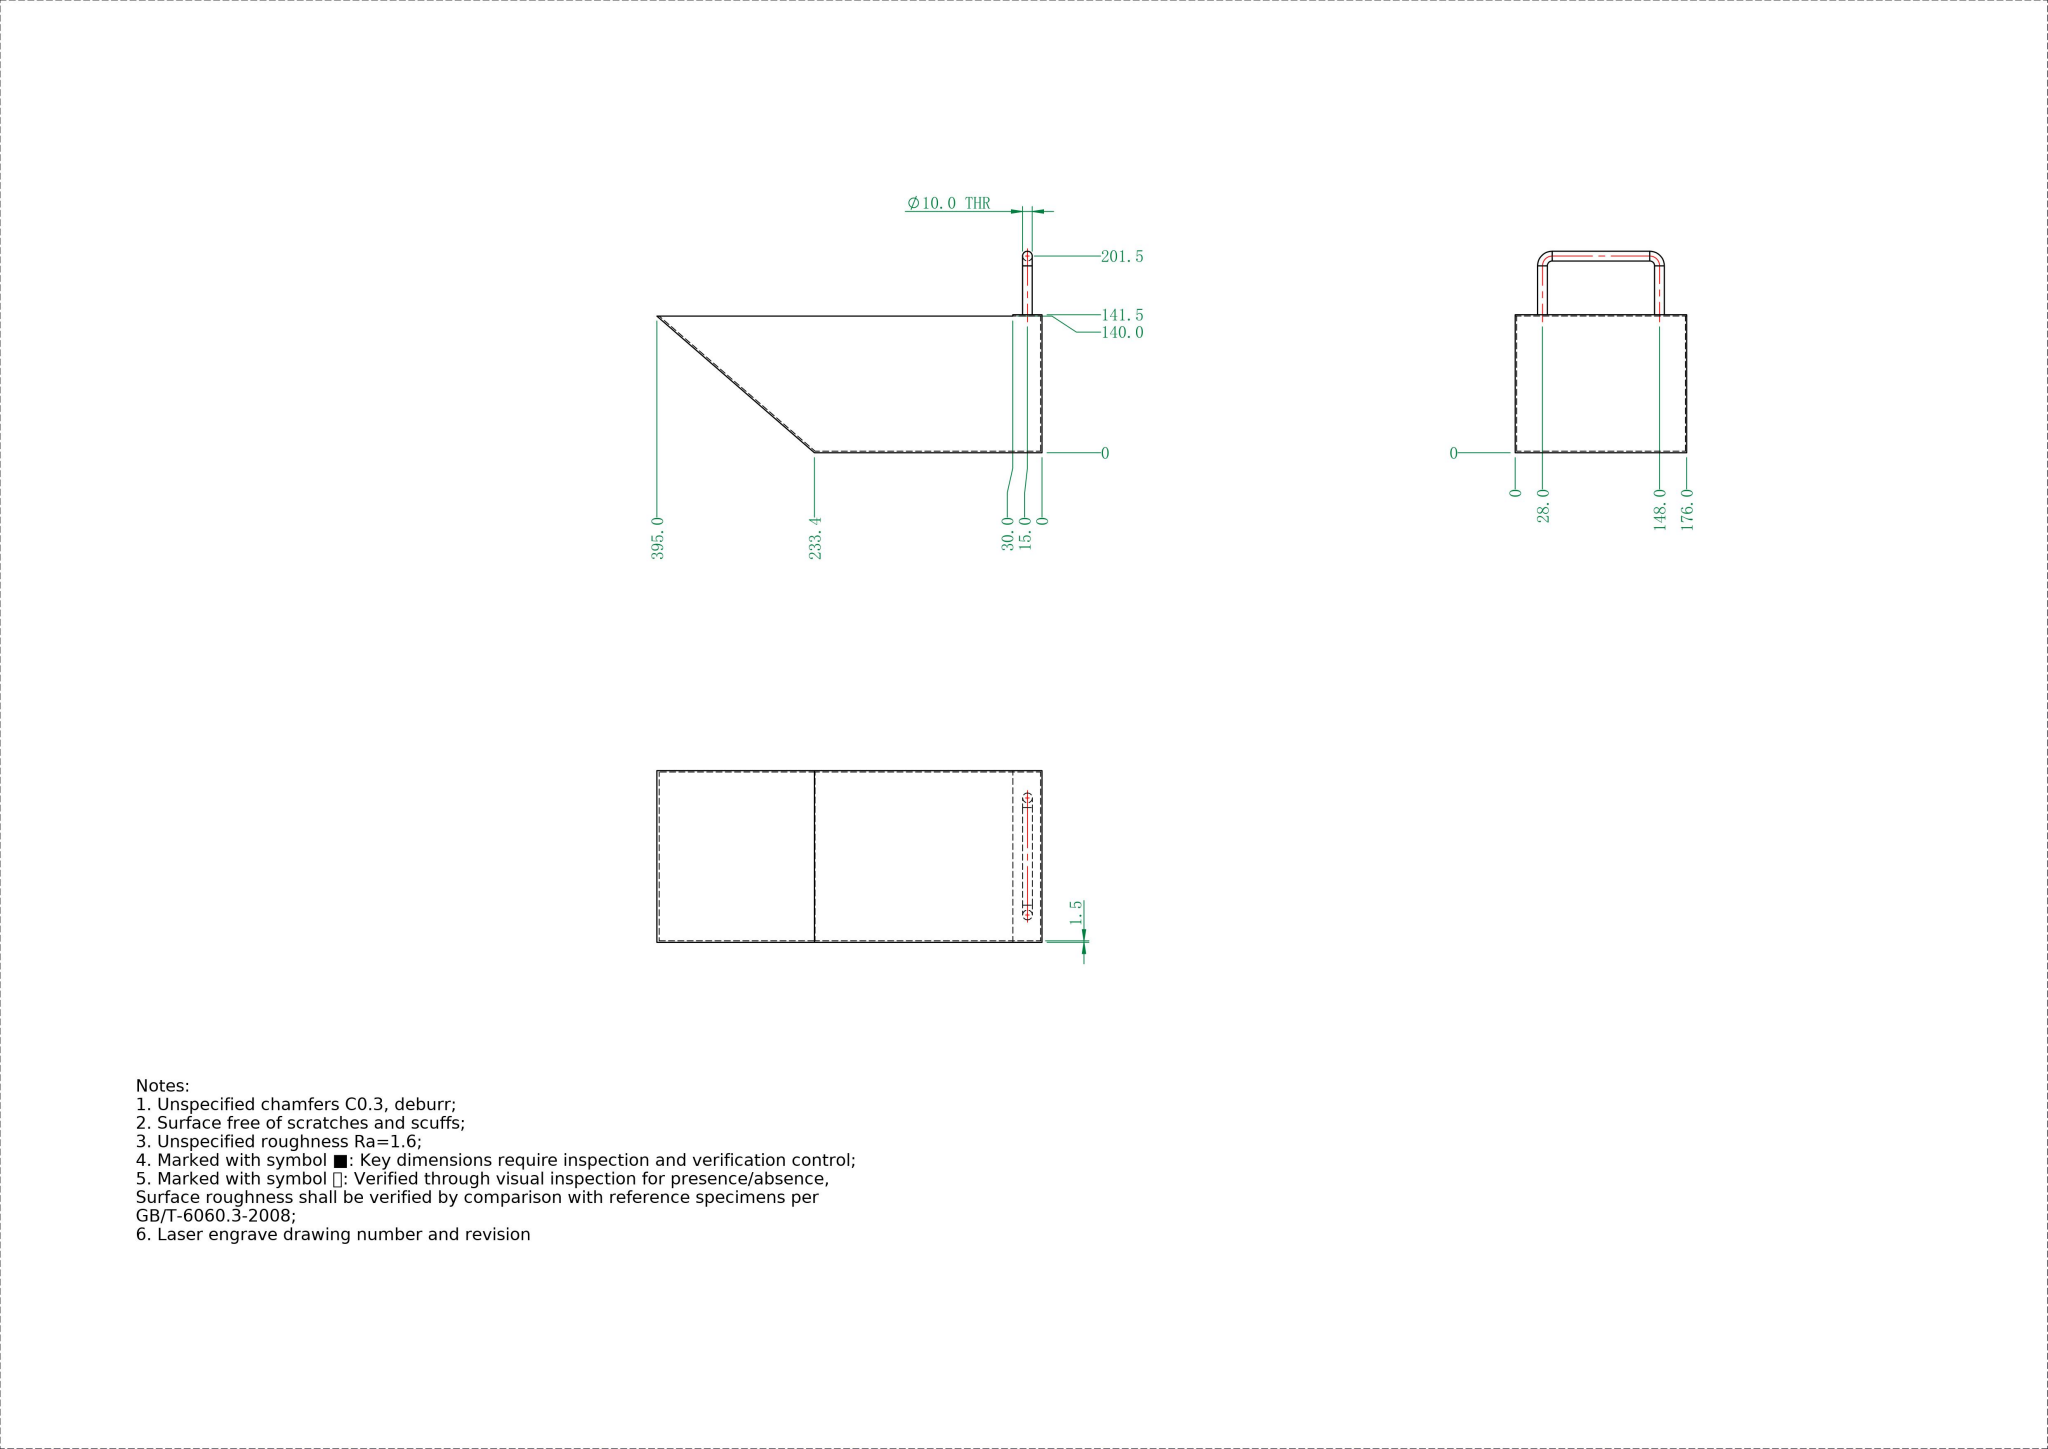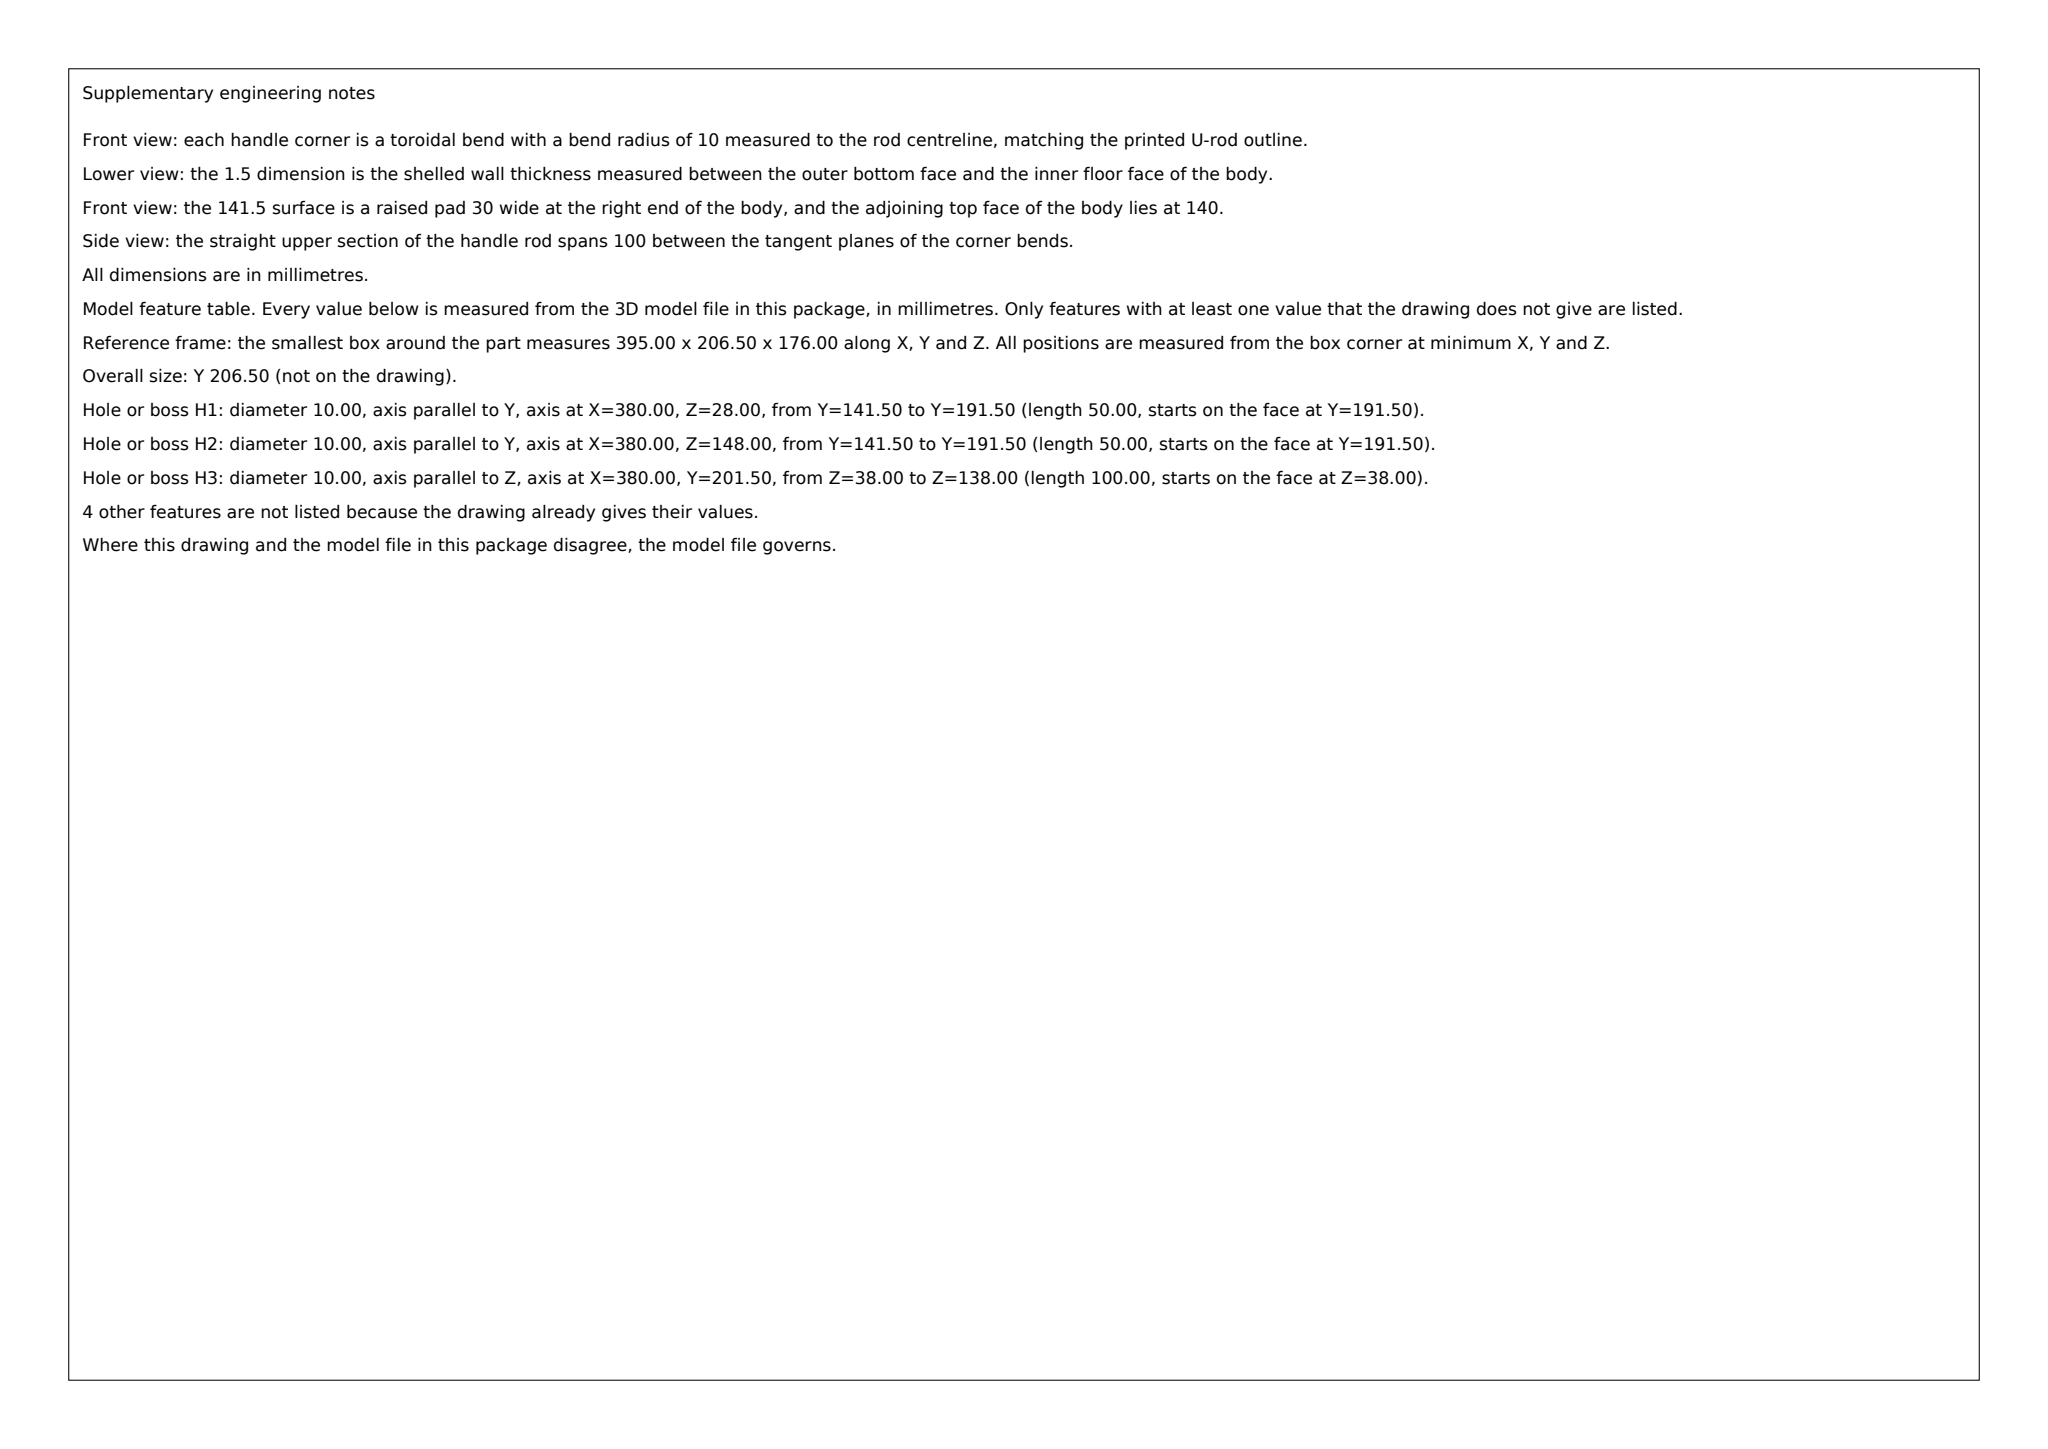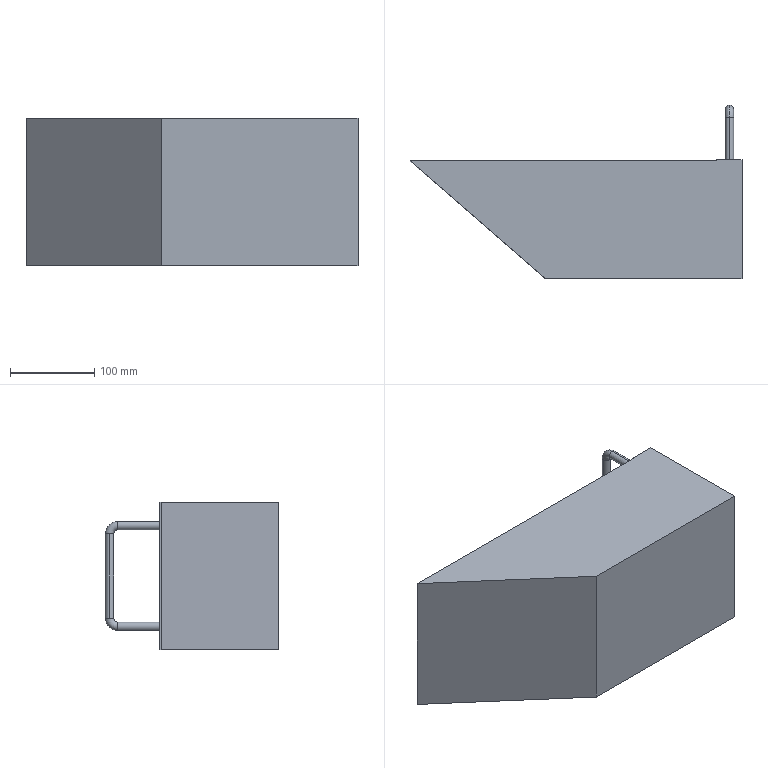Part | SolidWorks | mm | 1 solid | 24 faces | box 395 x 206.5 x 176 mm | volume 309691 mm3 | plane 14 | cylinder 6 | torus 4 | commonest cylinder face diameters 10 x6
Drawing notes:
Ø10.0 THRU | from the solid: Three Ø10.0 cylinders (y-axis at x380,z148 & x380,z28; z-axis at x380,y201.5) all full-depth, dia 10.0
STEP:
#1=CARTESIAN_POINT('',(375.,201.5,38.));
#2=VERTEX_POINT('',#1);
#3=CARTESIAN_POINT('',(380.,206.5,38.));
#4=VERTEX_POINT('',#3);
#5=CARTESIAN_POINT('',(380.,201.5,38.));
#6=DIRECTION('',(0.,0.,-1.));
#7=DIRECTION('',(0.,1.,0.));
#8=AXIS2_PLACEMENT_3D('',#5,#6,#7);
#9=CIRCLE('',#8,5.);
#10=EDGE_CURVE('',#2,#4,#9,.T.);
#11=ORIENTED_EDGE('',*,*,#10,.T.);
#12=CARTESIAN_POINT('',(380.,191.5,23.));
#13=VERTEX_POINT('',#12);
#14=CARTESIAN_POINT('',(380.,191.5,38.));
#15=DIRECTION('',(-1.,0.,0.));
#16=DIRECTION('',(0.,0.,1.));
#17=AXIS2_PLACEMENT_3D('',#14,#15,#16);
#18=CIRCLE('',#17,15.);
#19=EDGE_CURVE('',#4,#13,#18,.T.);
#20=ORIENTED_EDGE('',*,*,#19,.T.);
#21=CARTESIAN_POINT('',(380.,191.5,33.));
#22=VERTEX_POINT('',#21);
#23=CARTESIAN_POINT('',(380.,191.5,28.));
#24=DIRECTION('',(0.,-1.,0.));
#25=DIRECTION('',(0.,0.,-1.));
#26=AXIS2_PLACEMENT_3D('',#23,#24,#25);
#27=CIRCLE('',#26,5.);
#28=EDGE_CURVE('',#22,#13,#27,.T.);
#29=ORIENTED_EDGE('',*,*,#28,.F.);
#30=CARTESIAN_POINT('',(380.,196.5,38.));
#31=VERTEX_POINT('',#30);
#32=CARTESIAN_POINT('',(380.,191.5,38.));
#33=DIRECTION('',(-1.,0.,0.));
#34=DIRECTION('',(0.,0.,1.));
#35=AXIS2_PLACEMENT_3D('',#32,#33,#34);
#36=CIRCLE('',#35,5.);
#37=EDGE_CURVE('',#31,#22,#36,.T.);
#38=ORIENTED_EDGE('',*,*,#37,.F.);
#39=CARTESIAN_POINT('',(380.,201.5,38.));
#40=DIRECTION('',(0.,0.,-1.));
#41=DIRECTION('',(0.,1.,0.));
#42=AXIS2_PLACEMENT_3D('',#39,#40,#41);
#43=CIRCLE('',#42,5.);
#44=EDGE_CURVE('',#31,#2,#43,.T.);
#45=ORIENTED_EDGE('',*,*,#44,.T.);
#46=EDGE_LOOP('',(#11,#20,#29,#38,#45));
#47=FACE_OUTER_BOUND('',#46,.T.);
#48=CARTESIAN_POINT('',(380.,191.5,38.));
#49=DIRECTION('',(-1.,0.,0.));
#50=DIRECTION('',(0.,0.,1.));
#51=AXIS2_PLACEMENT_3D('',#48,#49,#50);
#52=TOROIDAL_SURFACE('',#51,10.,5.);
#53=ADVANCED_FACE('',(#47),#52,.T.);
#54=CARTESIAN_POINT('',(380.,191.5,143.));
#55=VERTEX_POINT('',#54);
#56=CARTESIAN_POINT('',(380.,191.5,153.));
#57=VERTEX_POINT('',#56);
#58=CARTESIAN_POINT('',(380.,191.5,148.));
#59=DIRECTION('',(0.,1.,0.));
#60=DIRECTION('',(0.,0.,1.));
#61=AXIS2_PLACEMENT_3D('',#58,#59,#60);
#62=CIRCLE('',#61,5.);
#63=EDGE_CURVE('',#55,#57,#62,.T.);
#64=ORIENTED_EDGE('',*,*,#63,.T.);
#65=CARTESIAN_POINT('',(380.,206.5,138.));
#66=VERTEX_POINT('',#65);
#67=CARTESIAN_POINT('',(380.,191.5,138.));
#68=DIRECTION('',(-1.,0.,0.));
#69=DIRECTION('',(0.,0.,1.));
#70=AXIS2_PLACEMENT_3D('',#67,#68,#69);
#71=CIRCLE('',#70,15.);
#72=EDGE_CURVE('',#57,#66,#71,.T.);
#73=ORIENTED_EDGE('',*,*,#72,.T.);
#74=CARTESIAN_POINT('',(375.,201.5,138.));
#75=VERTEX_POINT('',#74);
#76=CARTESIAN_POINT('',(380.,201.5,138.));
#77=DIRECTION('',(0.,0.,-1.));
#78=DIRECTION('',(0.,1.,0.));
#79=AXIS2_PLACEMENT_3D('',#76,#77,#78);
#80=CIRCLE('',#79,5.);
#81=EDGE_CURVE('',#75,#66,#80,.T.);
#82=ORIENTED_EDGE('',*,*,#81,.F.);
#83=CARTESIAN_POINT('',(380.,196.5,138.));
#84=VERTEX_POINT('',#83);
#85=CARTESIAN_POINT('',(380.,201.5,138.));
#86=DIRECTION('',(0.,0.,-1.));
#87=DIRECTION('',(0.,1.,0.));
#88=AXIS2_PLACEMENT_3D('',#85,#86,#87);
#89=CIRCLE('',#88,5.);
#90=EDGE_CURVE('',#84,#75,#89,.T.);
#91=ORIENTED_EDGE('',*,*,#90,.F.);
#92=CARTESIAN_POINT('',(380.,191.5,138.));
#93=DIRECTION('',(-1.,0.,0.));
#94=DIRECTION('',(0.,0.,1.));
#95=AXIS2_PLACEMENT_3D('',#92,#93,#94);
#96=CIRCLE('',#95,5.);
#97=EDGE_CURVE('',#55,#84,#96,.T.);
#98=ORIENTED_EDGE('',*,*,#97,.F.);
#99=EDGE_LOOP('',(#64,#73,#82,#91,#98));
#100=FACE_OUTER_BOUND('',#99,.T.);
#101=CARTESIAN_POINT('',(380.,191.5,138.));
#102=DIRECTION('',(-1.,0.,0.));
#103=DIRECTION('',(0.,0.,1.));
#104=AXIS2_PLACEMENT_3D('',#101,#102,#103);
#105=TOROIDAL_SURFACE('',#104,10.,5.);
#106=ADVANCED_FACE('',(#100),#105,.T.);
#107=CARTESIAN_POINT('',(380.,191.5,28.));
#108=DIRECTION('',(0.,-1.,0.));
#109=DIRECTION('',(0.,0.,-1.));
#110=AXIS2_PLACEMENT_3D('',#107,#108,#109);
#111=CIRCLE('',#110,5.);
#112=EDGE_CURVE('',#13,#22,#111,.T.);
#113=ORIENTED_EDGE('',*,*,#112,.T.);
#114=CARTESIAN_POINT('',(380.,141.5,33.));
#115=VERTEX_POINT('',#114);
#116=CARTESIAN_POINT('',(380.,191.5,33.));
#117=DIRECTION('',(0.,-1.,-0.));
#118=VECTOR('',#117,1000.);
#119=LINE('',#116,#118);
#120=EDGE_CURVE('',#22,#115,#119,.T.);
#121=ORIENTED_EDGE('',*,*,#120,.T.);
#122=CARTESIAN_POINT('',(380.,141.5,23.));
#123=VERTEX_POINT('',#122);
#124=CARTESIAN_POINT('',(380.,141.5,28.));
#125=DIRECTION('',(0.,-1.,-0.));
#126=DIRECTION('',(0.,0.,-1.));
#127=AXIS2_PLACEMENT_3D('',#124,#125,#126);
#128=CIRCLE('',#127,5.);
#129=EDGE_CURVE('',#123,#115,#128,.T.);
#130=ORIENTED_EDGE('',*,*,#129,.F.);
#131=CARTESIAN_POINT('',(380.,191.5,23.));
#132=DIRECTION('',(0.,-1.,-0.));
#133=VECTOR('',#132,1000.);
#134=LINE('',#131,#133);
#135=EDGE_CURVE('',#13,#123,#134,.T.);
#136=ORIENTED_EDGE('',*,*,#135,.F.);
#137=EDGE_LOOP('',(#113,#121,#130,#136));
#138=FACE_OUTER_BOUND('',#137,.T.);
#139=CARTESIAN_POINT('',(380.,191.5,28.));
#140=DIRECTION('',(0.,-1.,-0.));
#141=DIRECTION('',(0.,0.,-1.));
#142=AXIS2_PLACEMENT_3D('',#139,#140,#141);
#143=CYLINDRICAL_SURFACE('',#142,5.);
#144=ADVANCED_FACE('',(#138),#143,.T.);
#145=ORIENTED_EDGE('',*,*,#81,.T.);
#146=CARTESIAN_POINT('',(385.,201.5,138.));
#147=VERTEX_POINT('',#146);
#148=CARTESIAN_POINT('',(380.,201.5,138.));
#149=DIRECTION('',(0.,0.,-1.));
#150=DIRECTION('',(0.,1.,0.));
#151=AXIS2_PLACEMENT_3D('',#148,#149,#150);
#152=CIRCLE('',#151,5.);
#153=EDGE_CURVE('',#66,#147,#152,.T.);
#154=ORIENTED_EDGE('',*,*,#153,.T.);
#155=CARTESIAN_POINT('',(385.,201.5,38.));
#156=VERTEX_POINT('',#155);
#157=CARTESIAN_POINT('',(385.,201.5,138.));
#158=DIRECTION('',(0.,0.,-1.));
#159=VECTOR('',#158,1000.);
#160=LINE('',#157,#159);
#161=EDGE_CURVE('',#147,#156,#160,.T.);
#162=ORIENTED_EDGE('',*,*,#161,.T.);
#163=CARTESIAN_POINT('',(380.,201.5,38.));
#164=DIRECTION('',(0.,0.,-1.));
#165=DIRECTION('',(0.,1.,0.));
#166=AXIS2_PLACEMENT_3D('',#163,#164,#165);
#167=CIRCLE('',#166,5.);
#168=EDGE_CURVE('',#4,#156,#167,.T.);
#169=ORIENTED_EDGE('',*,*,#168,.F.);
#170=ORIENTED_EDGE('',*,*,#10,.F.);
#171=CARTESIAN_POINT('',(375.,201.5,138.));
#172=DIRECTION('',(0.,0.,-1.));
#173=VECTOR('',#172,1000.);
#174=LINE('',#171,#173);
#175=EDGE_CURVE('',#75,#2,#174,.T.);
#176=ORIENTED_EDGE('',*,*,#175,.F.);
#177=EDGE_LOOP('',(#145,#154,#162,#169,#170,#176));
#178=FACE_OUTER_BOUND('',#177,.T.);
#179=CARTESIAN_POINT('',(380.,201.5,138.));
#180=DIRECTION('',(0.,0.,-1.));
#181=DIRECTION('',(-1.,0.,0.));
#182=AXIS2_PLACEMENT_3D('',#179,#180,#181);
#183=CYLINDRICAL_SURFACE('',#182,5.);
#184=ADVANCED_FACE('',(#178),#183,.T.);
#185=CARTESIAN_POINT('',(380.,141.5,153.));
#186=VERTEX_POINT('',#185);
#187=CARTESIAN_POINT('',(380.,141.5,143.));
#188=VERTEX_POINT('',#187);
#189=CARTESIAN_POINT('',(380.,141.5,148.));
#190=DIRECTION('',(0.,1.,0.));
#191=DIRECTION('',(0.,0.,1.));
#192=AXIS2_PLACEMENT_3D('',#189,#190,#191);
#193=CIRCLE('',#192,5.);
#194=EDGE_CURVE('',#186,#188,#193,.T.);
#195=ORIENTED_EDGE('',*,*,#194,.T.);
#196=CARTESIAN_POINT('',(380.,141.5,143.));
#197=DIRECTION('',(0.,1.,0.));
#198=VECTOR('',#197,1000.);
#199=LINE('',#196,#198);
#200=EDGE_CURVE('',#188,#55,#199,.T.);
#201=ORIENTED_EDGE('',*,*,#200,.T.);
#202=CARTESIAN_POINT('',(380.,191.5,148.));
#203=DIRECTION('',(0.,1.,0.));
#204=DIRECTION('',(0.,0.,1.));
#205=AXIS2_PLACEMENT_3D('',#202,#203,#204);
#206=CIRCLE('',#205,5.);
#207=EDGE_CURVE('',#57,#55,#206,.T.);
#208=ORIENTED_EDGE('',*,*,#207,.F.);
#209=CARTESIAN_POINT('',(380.,141.5,153.));
#210=DIRECTION('',(0.,1.,0.));
#211=VECTOR('',#210,1000.);
#212=LINE('',#209,#211);
#213=EDGE_CURVE('',#186,#57,#212,.T.);
#214=ORIENTED_EDGE('',*,*,#213,.F.);
#215=EDGE_LOOP('',(#195,#201,#208,#214));
#216=FACE_OUTER_BOUND('',#215,.T.);
#217=CARTESIAN_POINT('',(380.,141.5,148.));
#218=DIRECTION('',(0.,1.,0.));
#219=DIRECTION('',(0.,0.,1.));
#220=AXIS2_PLACEMENT_3D('',#217,#218,#219);
#221=CYLINDRICAL_SURFACE('',#220,5.);
#222=ADVANCED_FACE('',(#216),#221,.T.);
#223=CARTESIAN_POINT('',(395.,141.5,176.));
#224=VERTEX_POINT('',#223);
#225=CARTESIAN_POINT('',(395.,141.5,0.));
#226=VERTEX_POINT('',#225);
#227=CARTESIAN_POINT('',(395.,141.5,0.));
#228=DIRECTION('',(0.,0.,-1.));
#229=VECTOR('',#228,1000.);
#230=LINE('',#227,#229);
#231=EDGE_CURVE('',#224,#226,#230,.T.);
#232=ORIENTED_EDGE('',*,*,#231,.T.);
#233=CARTESIAN_POINT('',(365.,141.5,0.));
#234=VERTEX_POINT('',#233);
#235=CARTESIAN_POINT('',(395.,141.5,0.));
#236=DIRECTION('',(-1.,0.,0.));
#237=VECTOR('',#236,1000.);
#238=LINE('',#235,#237);
#239=EDGE_CURVE('',#226,#234,#238,.T.);
#240=ORIENTED_EDGE('',*,*,#239,.T.);
#241=CARTESIAN_POINT('',(365.,141.5,176.));
#242=VERTEX_POINT('',#241);
#243=CARTESIAN_POINT('',(365.,141.5,0.));
#244=DIRECTION('',(0.,0.,1.));
#245=VECTOR('',#244,1000.);
#246=LINE('',#243,#245);
#247=EDGE_CURVE('',#234,#242,#246,.T.);
#248=ORIENTED_EDGE('',*,*,#247,.T.);
#249=CARTESIAN_POINT('',(395.,141.5,176.));
#250=DIRECTION('',(1.,0.,0.));
#251=VECTOR('',#250,1000.);
#252=LINE('',#249,#251);
#253=EDGE_CURVE('',#242,#224,#252,.T.);
#254=ORIENTED_EDGE('',*,*,#253,.T.);
#255=EDGE_LOOP('',(#232,#240,#248,#254));
#256=FACE_OUTER_BOUND('',#255,.T.);
#257=ORIENTED_EDGE('',*,*,#194,.F.);
#258=CARTESIAN_POINT('',(380.,141.5,148.));
#259=DIRECTION('',(0.,1.,0.));
#260=DIRECTION('',(0.,0.,1.));
#261=AXIS2_PLACEMENT_3D('',#258,#259,#260);
#262=CIRCLE('',#261,5.);
#263=EDGE_CURVE('',#188,#186,#262,.T.);
#264=ORIENTED_EDGE('',*,*,#263,.F.);
#265=EDGE_LOOP('',(#257,#264));
#266=FACE_BOUND('',#265,.T.);
#267=ORIENTED_EDGE('',*,*,#129,.T.);
#268=CARTESIAN_POINT('',(380.,141.5,28.));
#269=DIRECTION('',(0.,-1.,-0.));
#270=DIRECTION('',(0.,0.,-1.));
#271=AXIS2_PLACEMENT_3D('',#268,#269,#270);
#272=CIRCLE('',#271,5.);
#273=EDGE_CURVE('',#115,#123,#272,.T.);
#274=ORIENTED_EDGE('',*,*,#273,.T.);
#275=EDGE_LOOP('',(#267,#274));
#276=FACE_BOUND('',#275,.T.);
#277=CARTESIAN_POINT('',(0.,141.5,0.));
#278=DIRECTION('',(0.,-1.,0.));
#279=DIRECTION('',(0.,0.,-1.));
#280=AXIS2_PLACEMENT_3D('',#277,#278,#279);
#281=PLANE('',#280);
#282=ADVANCED_FACE('',(#256,#266,#276),#281,.F.);
#283=CARTESIAN_POINT('',(365.,140.,0.));
#284=VERTEX_POINT('',#283);
#285=CARTESIAN_POINT('',(365.,140.,1.5));
#286=VERTEX_POINT('',#285);
#287=CARTESIAN_POINT('',(365.,140.,0.));
#288=DIRECTION('',(0.,0.,1.));
#289=VECTOR('',#288,1000.);
#290=LINE('',#287,#289);
#291=EDGE_CURVE('',#284,#286,#290,.T.);
#292=ORIENTED_EDGE('',*,*,#291,.F.);
#293=CARTESIAN_POINT('',(0.,140.,0.));
#294=VERTEX_POINT('',#293);
#295=CARTESIAN_POINT('',(0.,140.,0.));
#296=DIRECTION('',(-1.,0.,0.));
#297=VECTOR('',#296,1000.);
#298=LINE('',#295,#297);
#299=EDGE_CURVE('',#284,#294,#298,.T.);
#300=ORIENTED_EDGE('',*,*,#299,.T.);
#301=CARTESIAN_POINT('',(0.,140.,176.));
#302=VERTEX_POINT('',#301);
#303=CARTESIAN_POINT('',(0.,140.,176.));
#304=DIRECTION('',(0.,0.,-1.));
#305=VECTOR('',#304,1000.);
#306=LINE('',#303,#305);
#307=EDGE_CURVE('',#302,#294,#306,.T.);
#308=ORIENTED_EDGE('',*,*,#307,.F.);
#309=CARTESIAN_POINT('',(365.,140.,176.));
#310=VERTEX_POINT('',#309);
#311=CARTESIAN_POINT('',(0.,140.,176.));
#312=DIRECTION('',(-1.,0.,0.));
#313=VECTOR('',#312,1000.);
#314=LINE('',#311,#313);
#315=EDGE_CURVE('',#310,#302,#314,.T.);
#316=ORIENTED_EDGE('',*,*,#315,.F.);
#317=CARTESIAN_POINT('',(365.,140.,174.5));
#318=VERTEX_POINT('',#317);
#319=CARTESIAN_POINT('',(365.,140.,0.));
#320=DIRECTION('',(0.,0.,1.));
#321=VECTOR('',#320,1000.);
#322=LINE('',#319,#321);
#323=EDGE_CURVE('',#318,#310,#322,.T.);
#324=ORIENTED_EDGE('',*,*,#323,.F.);
#325=CARTESIAN_POINT('',(2.291,140.,174.5));
#326=VERTEX_POINT('',#325);
#327=CARTESIAN_POINT('',(0.,140.,174.5));
#328=DIRECTION('',(-1.,0.,0.));
#329=VECTOR('',#328,1000.);
#330=LINE('',#327,#329);
#331=EDGE_CURVE('',#318,#326,#330,.T.);
#332=ORIENTED_EDGE('',*,*,#331,.T.);
#333=CARTESIAN_POINT('',(2.291,140.,1.5));
#334=VERTEX_POINT('',#333);
#335=CARTESIAN_POINT('',(2.291,140.,-15.));
#336=DIRECTION('',(0.,0.,-1.));
#337=VECTOR('',#336,1000.);
#338=LINE('',#335,#337);
#339=EDGE_CURVE('',#326,#334,#338,.T.);
#340=ORIENTED_EDGE('',*,*,#339,.T.);
#341=CARTESIAN_POINT('',(0.,140.,1.5));
#342=DIRECTION('',(-1.,0.,0.));
#343=VECTOR('',#342,1000.);
#344=LINE('',#341,#343);
#345=EDGE_CURVE('',#286,#334,#344,.T.);
#346=ORIENTED_EDGE('',*,*,#345,.F.);
#347=EDGE_LOOP('',(#292,#300,#308,#316,#324,#332,#340,#346));
#348=FACE_OUTER_BOUND('',#347,.T.);
#349=CARTESIAN_POINT('',(0.,140.,176.));
#350=DIRECTION('',(0.,-1.,0.));
#351=DIRECTION('',(0.,0.,-1.));
#352=AXIS2_PLACEMENT_3D('',#349,#350,#351);
#353=PLANE('',#352);
#354=ADVANCED_FACE('',(#348),#353,.F.);
#355=CARTESIAN_POINT('',(161.563,0.,176.));
#356=VERTEX_POINT('',#355);
#357=CARTESIAN_POINT('',(395.,0.,176.));
#358=VERTEX_POINT('',#357);
#359=CARTESIAN_POINT('',(0.,0.,176.));
#360=DIRECTION('',(1.,0.,0.));
#361=VECTOR('',#360,1000.);
#362=LINE('',#359,#361);
#363=EDGE_CURVE('',#356,#358,#362,.T.);
#364=ORIENTED_EDGE('',*,*,#363,.F.);
#365=CARTESIAN_POINT('',(161.563,0.,0.));
#366=VERTEX_POINT('',#365);
#367=CARTESIAN_POINT('',(161.563,0.,-15.));
#368=DIRECTION('',(0.,0.,1.));
#369=VECTOR('',#368,1000.);
#370=LINE('',#367,#369);
#371=EDGE_CURVE('',#366,#356,#370,.T.);
#372=ORIENTED_EDGE('',*,*,#371,.F.);
#373=CARTESIAN_POINT('',(395.,0.,0.));
#374=VERTEX_POINT('',#373);
#375=CARTESIAN_POINT('',(0.,0.,0.));
#376=DIRECTION('',(1.,0.,0.));
#377=VECTOR('',#376,1000.);
#378=LINE('',#375,#377);
#379=EDGE_CURVE('',#366,#374,#378,.T.);
#380=ORIENTED_EDGE('',*,*,#379,.T.);
#381=CARTESIAN_POINT('',(395.,0.,176.));
#382=DIRECTION('',(0.,0.,-1.));
#383=VECTOR('',#382,1000.);
#384=LINE('',#381,#383);
#385=EDGE_CURVE('',#358,#374,#384,.T.);
#386=ORIENTED_EDGE('',*,*,#385,.F.);
#387=EDGE_LOOP('',(#364,#372,#380,#386));
#388=FACE_OUTER_BOUND('',#387,.T.);
#389=CARTESIAN_POINT('',(0.,0.,176.));
#390=DIRECTION('',(0.,1.,0.));
#391=DIRECTION('',(0.,0.,1.));
#392=AXIS2_PLACEMENT_3D('',#389,#390,#391);
#393=PLANE('',#392);
#394=ADVANCED_FACE('',(#388),#393,.F.);
#395=CARTESIAN_POINT('',(395.,0.,0.));
#396=DIRECTION('',(0.,1.,0.));
#397=VECTOR('',#396,1000.);
#398=LINE('',#395,#397);
#399=EDGE_CURVE('',#374,#226,#398,.T.);
#400=ORIENTED_EDGE('',*,*,#399,.T.);
#401=ORIENTED_EDGE('',*,*,#231,.F.);
#402=CARTESIAN_POINT('',(395.,0.,176.));
#403=DIRECTION('',(0.,1.,0.));
#404=VECTOR('',#403,1000.);
#405=LINE('',#402,#404);
#406=EDGE_CURVE('',#358,#224,#405,.T.);
#407=ORIENTED_EDGE('',*,*,#406,.F.);
#408=ORIENTED_EDGE('',*,*,#385,.T.);
#409=EDGE_LOOP('',(#400,#401,#407,#408));
#410=FACE_OUTER_BOUND('',#409,.T.);
#411=CARTESIAN_POINT('',(395.,0.,176.));
#412=DIRECTION('',(-1.,0.,0.));
#413=DIRECTION('',(0.,0.,1.));
#414=AXIS2_PLACEMENT_3D('',#411,#412,#413);
#415=PLANE('',#414);
#416=ADVANCED_FACE('',(#410),#415,.F.);
#417=ORIENTED_EDGE('',*,*,#406,.T.);
#418=ORIENTED_EDGE('',*,*,#253,.F.);
#419=CARTESIAN_POINT('',(365.,141.5,176.));
#420=DIRECTION('',(0.,-1.,0.));
#421=VECTOR('',#420,1000.);
#422=LINE('',#419,#421);
#423=EDGE_CURVE('',#242,#310,#422,.T.);
#424=ORIENTED_EDGE('',*,*,#423,.T.);
#425=ORIENTED_EDGE('',*,*,#315,.T.);
#426=CARTESIAN_POINT('',(161.563,0.,176.));
#427=DIRECTION('',(-0.7557,0.6549,0.));
#428=VECTOR('',#427,1000.);
#429=LINE('',#426,#428);
#430=EDGE_CURVE('',#356,#302,#429,.T.);
#431=ORIENTED_EDGE('',*,*,#430,.F.);
#432=ORIENTED_EDGE('',*,*,#363,.T.);
#433=EDGE_LOOP('',(#417,#418,#424,#425,#431,#432));
#434=FACE_OUTER_BOUND('',#433,.T.);
#435=CARTESIAN_POINT('',(0.,0.,176.));
#436=DIRECTION('',(0.,0.,-1.));
#437=DIRECTION('',(-1.,0.,0.));
#438=AXIS2_PLACEMENT_3D('',#435,#436,#437);
#439=PLANE('',#438);
#440=ADVANCED_FACE('',(#434),#439,.F.);
#441=CARTESIAN_POINT('',(69.288,79.96,0.));
#442=DIRECTION('',(0.7557,-0.6549,0.));
#443=VECTOR('',#442,1000.);
#444=LINE('',#441,#443);
#445=EDGE_CURVE('',#294,#366,#444,.T.);
#446=ORIENTED_EDGE('',*,*,#445,.F.);
#447=ORIENTED_EDGE('',*,*,#299,.F.);
#448=CARTESIAN_POINT('',(365.,141.5,0.));
#449=DIRECTION('',(0.,-1.,0.));
#450=VECTOR('',#449,1000.);
#451=LINE('',#448,#450);
#452=EDGE_CURVE('',#234,#284,#451,.T.);
#453=ORIENTED_EDGE('',*,*,#452,.F.);
#454=ORIENTED_EDGE('',*,*,#239,.F.);
#455=ORIENTED_EDGE('',*,*,#399,.F.);
#456=ORIENTED_EDGE('',*,*,#379,.F.);
#457=EDGE_LOOP('',(#446,#447,#453,#454,#455,#456));
#458=FACE_OUTER_BOUND('',#457,.T.);
#459=CARTESIAN_POINT('',(0.,0.,0.));
#460=DIRECTION('',(0.,0.,-1.));
#461=DIRECTION('',(-1.,0.,0.));
#462=AXIS2_PLACEMENT_3D('',#459,#460,#461);
#463=PLANE('',#462);
#464=ADVANCED_FACE('',(#458),#463,.T.);
#465=ORIENTED_EDGE('',*,*,#445,.T.);
#466=ORIENTED_EDGE('',*,*,#371,.T.);
#467=ORIENTED_EDGE('',*,*,#430,.T.);
#468=ORIENTED_EDGE('',*,*,#307,.T.);
#469=EDGE_LOOP('',(#465,#466,#467,#468));
#470=FACE_OUTER_BOUND('',#469,.T.);
#471=CARTESIAN_POINT('',(161.563,0.,-15.));
#472=DIRECTION('',(0.6549,0.7557,0.));
#473=DIRECTION('',(-0.7557,0.6549,0.));
#474=AXIS2_PLACEMENT_3D('',#471,#472,#473);
#475=PLANE('',#474);
#476=ADVANCED_FACE('',(#470),#475,.F.);
#477=CARTESIAN_POINT('',(162.123,1.5,174.5));
#478=VERTEX_POINT('',#477);
#479=CARTESIAN_POINT('',(393.5,1.5,174.5));
#480=VERTEX_POINT('',#479);
#481=CARTESIAN_POINT('',(0.,1.5,174.5));
#482=DIRECTION('',(1.,0.,0.));
#483=VECTOR('',#482,1000.);
#484=LINE('',#481,#483);
#485=EDGE_CURVE('',#478,#480,#484,.T.);
#486=ORIENTED_EDGE('',*,*,#485,.T.);
#487=CARTESIAN_POINT('',(393.5,1.5,1.5));
#488=VERTEX_POINT('',#487);
#489=CARTESIAN_POINT('',(393.5,1.5,176.));
#490=DIRECTION('',(0.,0.,-1.));
#491=VECTOR('',#490,1000.);
#492=LINE('',#489,#491);
#493=EDGE_CURVE('',#480,#488,#492,.T.);
#494=ORIENTED_EDGE('',*,*,#493,.T.);
#495=CARTESIAN_POINT('',(162.123,1.5,1.5));
#496=VERTEX_POINT('',#495);
#497=CARTESIAN_POINT('',(0.,1.5,1.5));
#498=DIRECTION('',(1.,0.,0.));
#499=VECTOR('',#498,1000.);
#500=LINE('',#497,#499);
#501=EDGE_CURVE('',#496,#488,#500,.T.);
#502=ORIENTED_EDGE('',*,*,#501,.F.);
#503=CARTESIAN_POINT('',(162.123,1.5,-15.));
#504=DIRECTION('',(0.,0.,1.));
#505=VECTOR('',#504,1000.);
#506=LINE('',#503,#505);
#507=EDGE_CURVE('',#496,#478,#506,.T.);
#508=ORIENTED_EDGE('',*,*,#507,.T.);
#509=EDGE_LOOP('',(#486,#494,#502,#508));
#510=FACE_OUTER_BOUND('',#509,.T.);
#511=CARTESIAN_POINT('',(0.,1.5,176.));
#512=DIRECTION('',(0.,1.,0.));
#513=DIRECTION('',(0.,0.,1.));
#514=AXIS2_PLACEMENT_3D('',#511,#512,#513);
#515=PLANE('',#514);
#516=ADVANCED_FACE('',(#510),#515,.T.);
#517=CARTESIAN_POINT('',(393.5,140.,1.5));
#518=VERTEX_POINT('',#517);
#519=CARTESIAN_POINT('',(393.5,0.,1.5));
#520=DIRECTION('',(0.,1.,0.));
#521=VECTOR('',#520,1000.);
#522=LINE('',#519,#521);
#523=EDGE_CURVE('',#488,#518,#522,.T.);
#524=ORIENTED_EDGE('',*,*,#523,.F.);
#525=ORIENTED_EDGE('',*,*,#493,.F.);
#526=CARTESIAN_POINT('',(393.5,140.,174.5));
#527=VERTEX_POINT('',#526);
#528=CARTESIAN_POINT('',(393.5,0.,174.5));
#529=DIRECTION('',(0.,1.,0.));
#530=VECTOR('',#529,1000.);
#531=LINE('',#528,#530);
#532=EDGE_CURVE('',#480,#527,#531,.T.);
#533=ORIENTED_EDGE('',*,*,#532,.T.);
#534=CARTESIAN_POINT('',(393.5,140.,176.));
#535=DIRECTION('',(0.,0.,-1.));
#536=VECTOR('',#535,1000.);
#537=LINE('',#534,#536);
#538=EDGE_CURVE('',#527,#518,#537,.T.);
#539=ORIENTED_EDGE('',*,*,#538,.T.);
#540=EDGE_LOOP('',(#524,#525,#533,#539));
#541=FACE_OUTER_BOUND('',#540,.T.);
#542=CARTESIAN_POINT('',(393.5,0.,176.));
#543=DIRECTION('',(-1.,0.,0.));
#544=DIRECTION('',(0.,0.,1.));
#545=AXIS2_PLACEMENT_3D('',#542,#543,#544);
#546=PLANE('',#545);
#547=ADVANCED_FACE('',(#541),#546,.T.);
#548=CARTESIAN_POINT('',(0.,140.,174.5));
#549=DIRECTION('',(-1.,0.,0.));
#550=VECTOR('',#549,1000.);
#551=LINE('',#548,#550);
#552=EDGE_CURVE('',#527,#318,#551,.T.);
#553=ORIENTED_EDGE('',*,*,#552,.F.);
#554=ORIENTED_EDGE('',*,*,#532,.F.);
#555=ORIENTED_EDGE('',*,*,#485,.F.);
#556=CARTESIAN_POINT('',(162.546,1.134,174.5));
#557=DIRECTION('',(-0.7557,0.6549,0.));
#558=VECTOR('',#557,1000.);
#559=LINE('',#556,#558);
#560=EDGE_CURVE('',#478,#326,#559,.T.);
#561=ORIENTED_EDGE('',*,*,#560,.T.);
#562=ORIENTED_EDGE('',*,*,#331,.F.);
#563=EDGE_LOOP('',(#553,#554,#555,#561,#562));
#564=FACE_OUTER_BOUND('',#563,.T.);
#565=CARTESIAN_POINT('',(0.,0.,174.5));
#566=DIRECTION('',(0.,0.,-1.));
#567=DIRECTION('',(-1.,0.,0.));
#568=AXIS2_PLACEMENT_3D('',#565,#566,#567);
#569=PLANE('',#568);
#570=ADVANCED_FACE('',(#564),#569,.T.);
#571=CARTESIAN_POINT('',(70.27,81.093,1.5));
#572=DIRECTION('',(0.7557,-0.6549,0.));
#573=VECTOR('',#572,1000.);
#574=LINE('',#571,#573);
#575=EDGE_CURVE('',#334,#496,#574,.T.);
#576=ORIENTED_EDGE('',*,*,#575,.T.);
#577=ORIENTED_EDGE('',*,*,#501,.T.);
#578=ORIENTED_EDGE('',*,*,#523,.T.);
#579=CARTESIAN_POINT('',(0.,140.,1.5));
#580=DIRECTION('',(-1.,0.,0.));
#581=VECTOR('',#580,1000.);
#582=LINE('',#579,#581);
#583=EDGE_CURVE('',#518,#286,#582,.T.);
#584=ORIENTED_EDGE('',*,*,#583,.T.);
#585=ORIENTED_EDGE('',*,*,#345,.T.);
#586=EDGE_LOOP('',(#576,#577,#578,#584,#585));
#587=FACE_OUTER_BOUND('',#586,.T.);
#588=CARTESIAN_POINT('',(0.,0.,1.5));
#589=DIRECTION('',(0.,0.,-1.));
#590=DIRECTION('',(-1.,0.,0.));
#591=AXIS2_PLACEMENT_3D('',#588,#589,#590);
#592=PLANE('',#591);
#593=ADVANCED_FACE('',(#587),#592,.F.);
#594=ORIENTED_EDGE('',*,*,#575,.F.);
#595=ORIENTED_EDGE('',*,*,#339,.F.);
#596=ORIENTED_EDGE('',*,*,#560,.F.);
#597=ORIENTED_EDGE('',*,*,#507,.F.);
#598=EDGE_LOOP('',(#594,#595,#596,#597));
#599=FACE_OUTER_BOUND('',#598,.T.);
#600=CARTESIAN_POINT('',(162.546,1.134,-15.));
#601=DIRECTION('',(0.6549,0.7557,0.));
#602=DIRECTION('',(-0.7557,0.6549,0.));
#603=AXIS2_PLACEMENT_3D('',#600,#601,#602);
#604=PLANE('',#603);
#605=ADVANCED_FACE('',(#599),#604,.T.);
#606=ORIENTED_EDGE('',*,*,#583,.F.);
#607=ORIENTED_EDGE('',*,*,#538,.F.);
#608=ORIENTED_EDGE('',*,*,#552,.T.);
#609=CARTESIAN_POINT('',(365.,140.,0.));
#610=DIRECTION('',(0.,0.,1.));
#611=VECTOR('',#610,1000.);
#612=LINE('',#609,#611);
#613=EDGE_CURVE('',#286,#318,#612,.T.);
#614=ORIENTED_EDGE('',*,*,#613,.F.);
#615=EDGE_LOOP('',(#606,#607,#608,#614));
#616=FACE_OUTER_BOUND('',#615,.T.);
#617=CARTESIAN_POINT('',(0.,140.,0.));
#618=DIRECTION('',(0.,-1.,0.));
#619=DIRECTION('',(0.,0.,-1.));
#620=AXIS2_PLACEMENT_3D('',#617,#618,#619);
#621=PLANE('',#620);
#622=ADVANCED_FACE('',(#616),#621,.T.);
#623=ORIENTED_EDGE('',*,*,#291,.T.);
#624=ORIENTED_EDGE('',*,*,#613,.T.);
#625=ORIENTED_EDGE('',*,*,#323,.T.);
#626=ORIENTED_EDGE('',*,*,#423,.F.);
#627=ORIENTED_EDGE('',*,*,#247,.F.);
#628=ORIENTED_EDGE('',*,*,#452,.T.);
#629=EDGE_LOOP('',(#623,#624,#625,#626,#627,#628));
#630=FACE_OUTER_BOUND('',#629,.T.);
#631=CARTESIAN_POINT('',(365.,141.5,0.));
#632=DIRECTION('',(1.,0.,-0.));
#633=DIRECTION('',(-0.,0.,-1.));
#634=AXIS2_PLACEMENT_3D('',#631,#632,#633);
#635=PLANE('',#634);
#636=ADVANCED_FACE('',(#630),#635,.F.);
#637=ORIENTED_EDGE('',*,*,#120,.F.);
#638=ORIENTED_EDGE('',*,*,#28,.T.);
#639=ORIENTED_EDGE('',*,*,#135,.T.);
#640=ORIENTED_EDGE('',*,*,#273,.F.);
#641=EDGE_LOOP('',(#637,#638,#639,#640));
#642=FACE_OUTER_BOUND('',#641,.T.);
#643=CARTESIAN_POINT('',(380.,191.5,28.));
#644=DIRECTION('',(0.,-1.,-0.));
#645=DIRECTION('',(0.,0.,-1.));
#646=AXIS2_PLACEMENT_3D('',#643,#644,#645);
#647=CYLINDRICAL_SURFACE('',#646,5.);
#648=ADVANCED_FACE('',(#642),#647,.T.);
#649=ORIENTED_EDGE('',*,*,#19,.F.);
#650=ORIENTED_EDGE('',*,*,#168,.T.);
#651=CARTESIAN_POINT('',(380.,201.5,38.));
#652=DIRECTION('',(0.,0.,-1.));
#653=DIRECTION('',(0.,1.,0.));
#654=AXIS2_PLACEMENT_3D('',#651,#652,#653);
#655=CIRCLE('',#654,5.);
#656=EDGE_CURVE('',#156,#31,#655,.T.);
#657=ORIENTED_EDGE('',*,*,#656,.T.);
#658=ORIENTED_EDGE('',*,*,#37,.T.);
#659=ORIENTED_EDGE('',*,*,#112,.F.);
#660=EDGE_LOOP('',(#649,#650,#657,#658,#659));
#661=FACE_OUTER_BOUND('',#660,.T.);
#662=CARTESIAN_POINT('',(380.,191.5,38.));
#663=DIRECTION('',(-1.,0.,0.));
#664=DIRECTION('',(0.,0.,1.));
#665=AXIS2_PLACEMENT_3D('',#662,#663,#664);
#666=TOROIDAL_SURFACE('',#665,10.,5.);
#667=ADVANCED_FACE('',(#661),#666,.T.);
#668=ORIENTED_EDGE('',*,*,#161,.F.);
#669=CARTESIAN_POINT('',(380.,201.5,138.));
#670=DIRECTION('',(0.,0.,-1.));
#671=DIRECTION('',(0.,1.,0.));
#672=AXIS2_PLACEMENT_3D('',#669,#670,#671);
#673=CIRCLE('',#672,5.);
#674=EDGE_CURVE('',#147,#84,#673,.T.);
#675=ORIENTED_EDGE('',*,*,#674,.T.);
#676=ORIENTED_EDGE('',*,*,#90,.T.);
#677=ORIENTED_EDGE('',*,*,#175,.T.);
#678=ORIENTED_EDGE('',*,*,#44,.F.);
#679=ORIENTED_EDGE('',*,*,#656,.F.);
#680=EDGE_LOOP('',(#668,#675,#676,#677,#678,#679));
#681=FACE_OUTER_BOUND('',#680,.T.);
#682=CARTESIAN_POINT('',(380.,201.5,138.));
#683=DIRECTION('',(0.,0.,-1.));
#684=DIRECTION('',(-1.,0.,0.));
#685=AXIS2_PLACEMENT_3D('',#682,#683,#684);
#686=CYLINDRICAL_SURFACE('',#685,5.);
#687=ADVANCED_FACE('',(#681),#686,.T.);
#688=ORIENTED_EDGE('',*,*,#72,.F.);
#689=ORIENTED_EDGE('',*,*,#207,.T.);
#690=ORIENTED_EDGE('',*,*,#97,.T.);
#691=ORIENTED_EDGE('',*,*,#674,.F.);
#692=ORIENTED_EDGE('',*,*,#153,.F.);
#693=EDGE_LOOP('',(#688,#689,#690,#691,#692));
#694=FACE_OUTER_BOUND('',#693,.T.);
#695=CARTESIAN_POINT('',(380.,191.5,138.));
#696=DIRECTION('',(-1.,0.,0.));
#697=DIRECTION('',(0.,0.,1.));
#698=AXIS2_PLACEMENT_3D('',#695,#696,#697);
#699=TOROIDAL_SURFACE('',#698,10.,5.);
#700=ADVANCED_FACE('',(#694),#699,.T.);
#701=ORIENTED_EDGE('',*,*,#200,.F.);
#702=ORIENTED_EDGE('',*,*,#263,.T.);
#703=ORIENTED_EDGE('',*,*,#213,.T.);
#704=ORIENTED_EDGE('',*,*,#63,.F.);
#705=EDGE_LOOP('',(#701,#702,#703,#704));
#706=FACE_OUTER_BOUND('',#705,.T.);
#707=CARTESIAN_POINT('',(380.,141.5,148.));
#708=DIRECTION('',(0.,1.,0.));
#709=DIRECTION('',(0.,0.,1.));
#710=AXIS2_PLACEMENT_3D('',#707,#708,#709);
#711=CYLINDRICAL_SURFACE('',#710,5.);
#712=ADVANCED_FACE('',(#706),#711,.T.);
#713=CLOSED_SHELL('',(#53,#106,#144,#184,#222,#282,#354,#394,#416,#440,#464,#476,#516,#547,#570,#593,#605,#622,#636,#648,#667,#687,#700,#712));
#714=MANIFOLD_SOLID_BREP('',#713);
#715=CARTESIAN_POINT('',(0.,0.,0.));
#716=DIRECTION('',(0.,0.,1.));
#717=DIRECTION('',(1.,0.,0.));
#718=AXIS2_PLACEMENT_3D('',#715,#716,#717);
#719=(LENGTH_UNIT()NAMED_UNIT(*)SI_UNIT(.MILLI.,.METRE.));
#720=UNCERTAINTY_MEASURE_WITH_UNIT(LENGTH_MEASURE(0.00001),#719,'','');
#721=(NAMED_UNIT(*)PLANE_ANGLE_UNIT()SI_UNIT($,.RADIAN.));
#722=(NAMED_UNIT(*)SI_UNIT($,.STERADIAN.)SOLID_ANGLE_UNIT());
#723=(GEOMETRIC_REPRESENTATION_CONTEXT(3)GLOBAL_UNCERTAINTY_ASSIGNED_CONTEXT((#720))GLOBAL_UNIT_ASSIGNED_CONTEXT((#719,#721,#722))REPRESENTATION_CONTEXT('',''));
#724=ADVANCED_BREP_SHAPE_REPRESENTATION('',(#714,#718),#723);